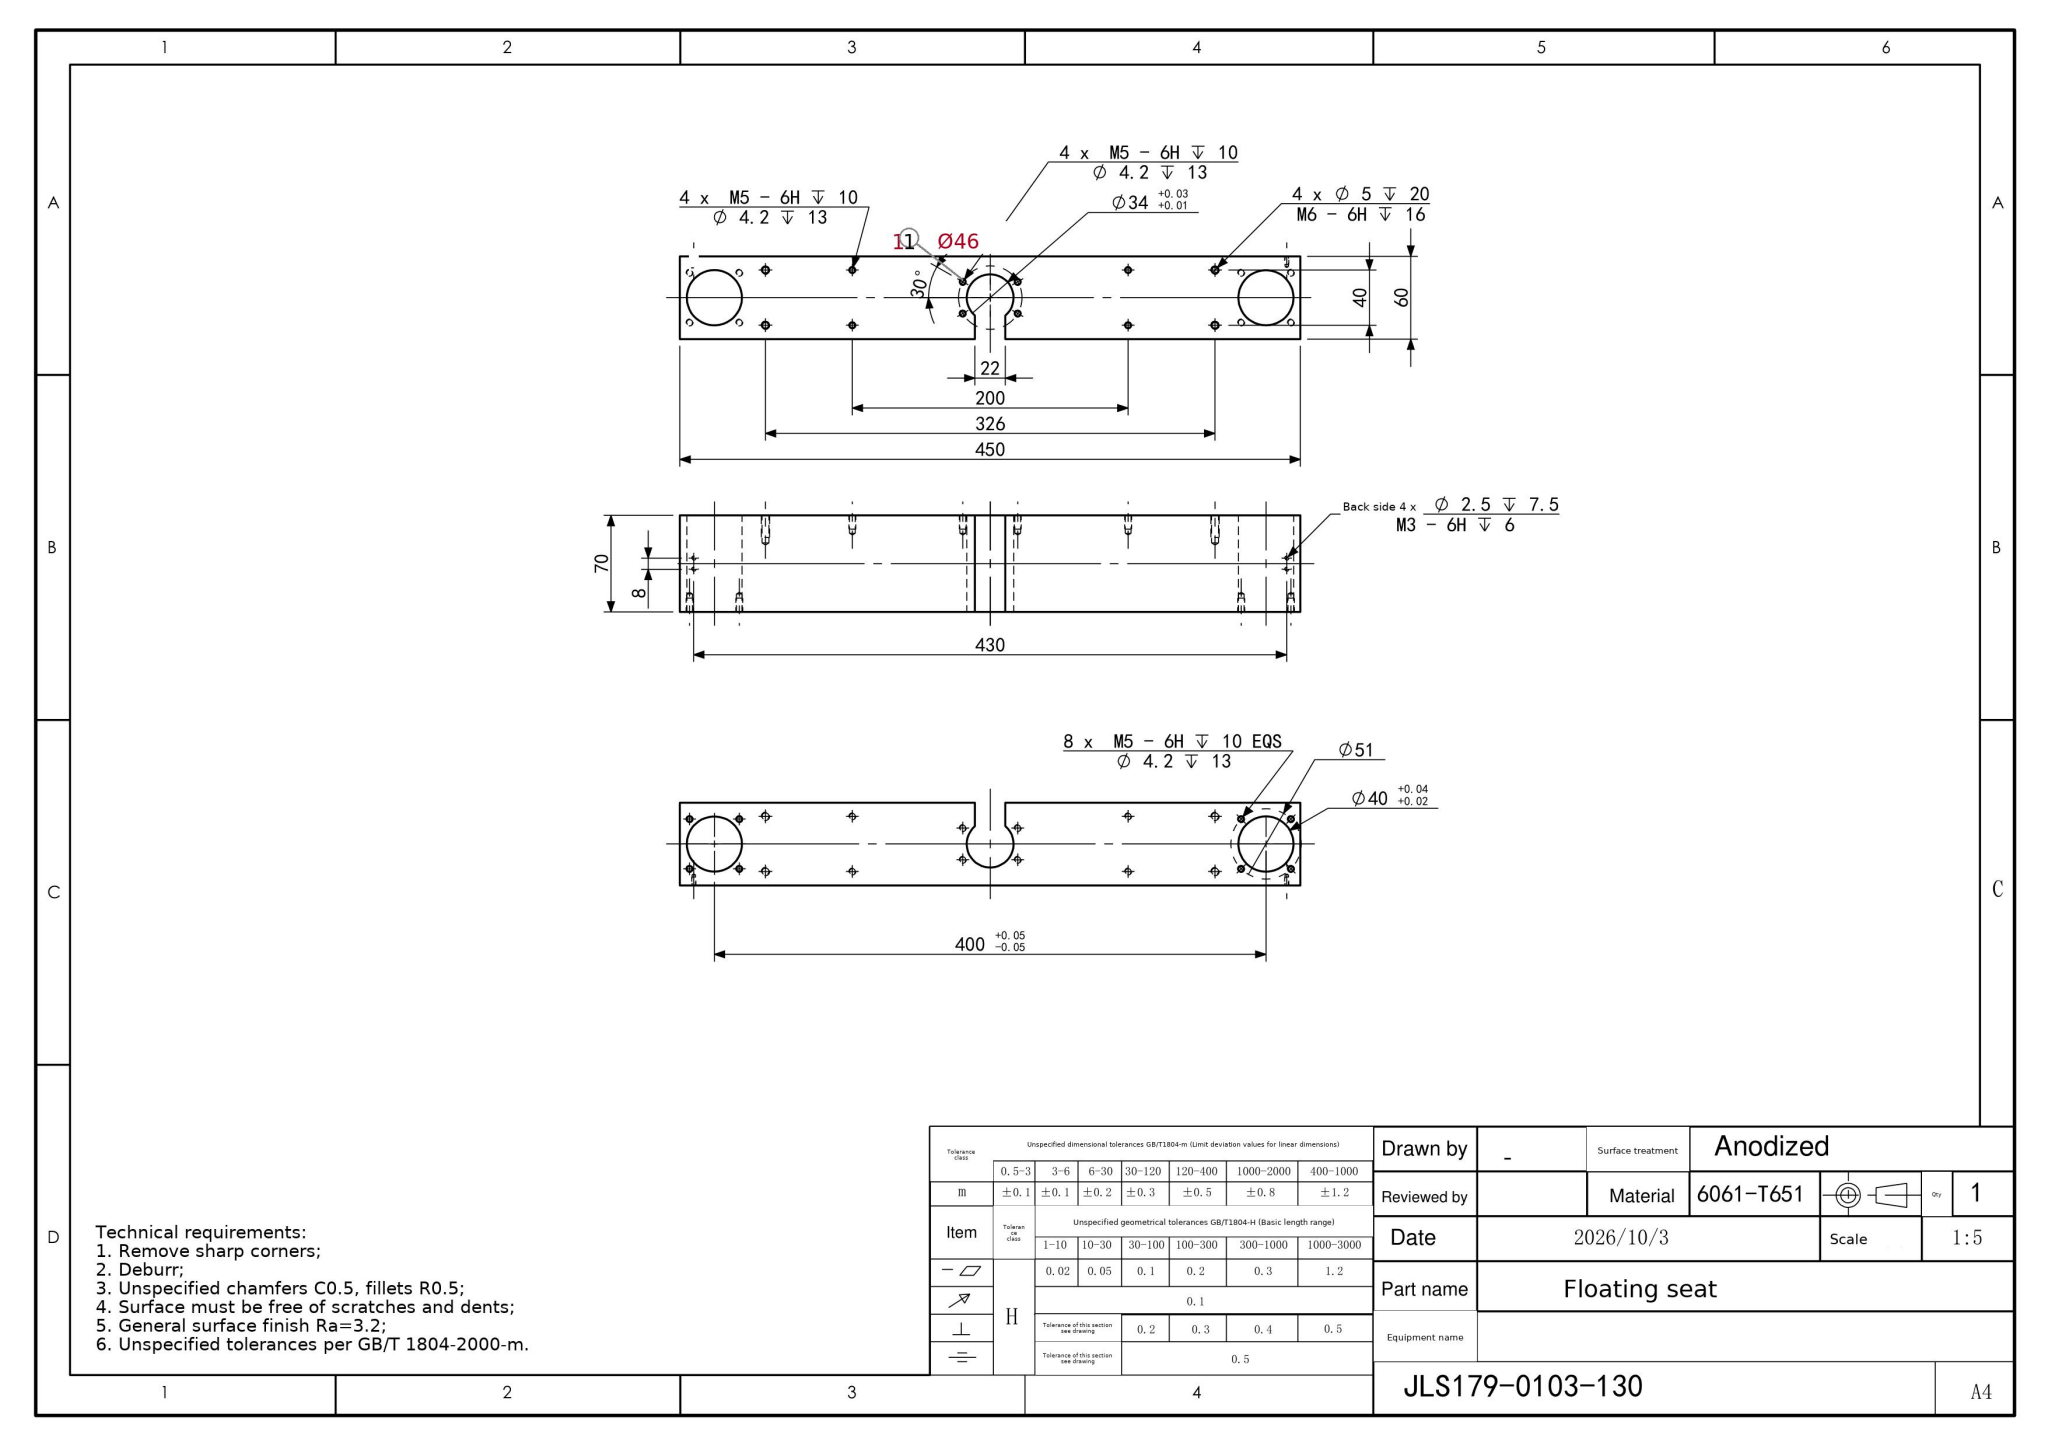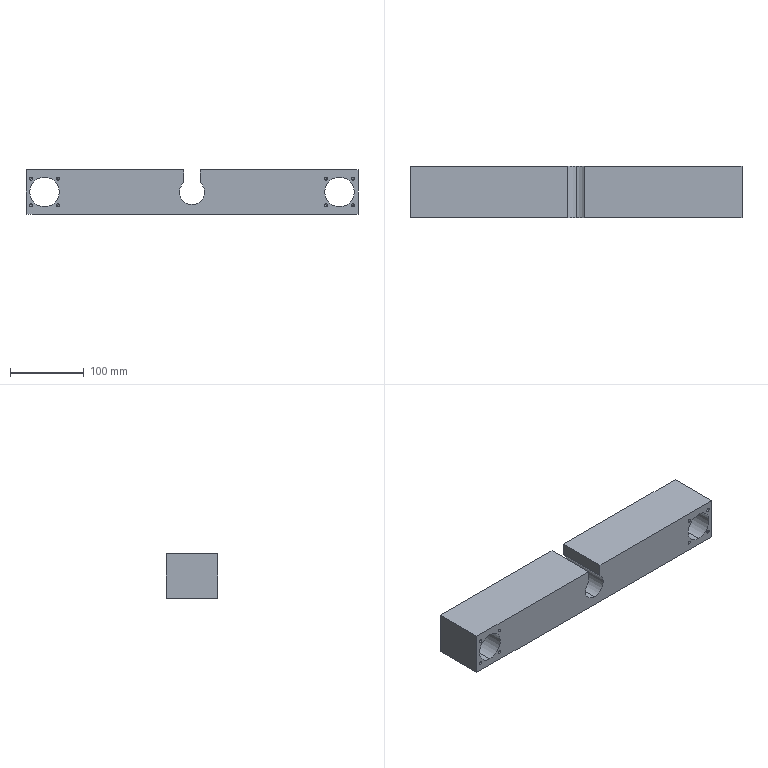Part | SolidWorks | mm | material 6061-T651 | 1 solid | 111 faces | box 450 x 70 x 60 mm | volume 1623796 mm3 | cylinder 54 | cone 48 | plane 9 | commonest cylinder face diameters 4.2 x32 2.5 x8 5 x8 40 x4 34 x2
build123d program:
from build123d import *

# Parameters (mm, degrees)
SKETCH1_W                  = 450
SKETCH1_H                  = 60
SKETCH1_R                  = 20
SKETCH1_R_2                = 17
BOSS_EXTRUDE1_DEPTH        = 35
M5_TAPPED_HOLE1_D          = 4.2
M5_TAPPED_HOLE1_DEPTH      = 13
M5_TAPPED_HOLE1_TIP        = 1.262
M6_TAPPED_HOLE2_D          = 5
M6_TAPPED_HOLE2_DEPTH      = 20
M6_TAPPED_HOLE2_TIP        = 1.502
M3_TAPPED_HOLE1_AT_2_COUNT = 2
M3_TAPPED_HOLE1_AT_2_PITCH = 8
SKETCH14_W                 = 22
SKETCH14_H                 = 121.424
CUT_EXTRUDE1_DEPTH         = 20
M5_TAPPED_HOLE2_D          = 4.2
M5_TAPPED_HOLE2_DEPTH      = 13
M5_TAPPED_HOLE2_TIP        = 1.262
M5_TAPPED_HOLE3_D          = 4.2
M5_TAPPED_HOLE3_DEPTH      = 13
M5_TAPPED_HOLE3_TIP        = 1.262


with BuildPart() as part:
    # Sketch1 → Boss-Extrude1 (new, symmetric)
    with BuildSketch(Plane(origin=(0, 0, 0), x_dir=(1, 0, 0), z_dir=(0, 1, 0))):
        Rectangle(SKETCH1_W, SKETCH1_H)
        with Locations(Location((200, 0, 0), (0, 0, 270))):
            Circle(SKETCH1_R, mode=Mode.SUBTRACT)
        with Locations(Location((-200, 0, 0), (0, 0, 90))):
            Circle(SKETCH1_R, mode=Mode.SUBTRACT)
        with Locations(Location((0, 0, 0), (0, 0, 270))):
            Circle(SKETCH1_R_2, mode=Mode.SUBTRACT)
    extrude(amount=BOSS_EXTRUDE1_DEPTH, both=True)

    # M5 Tapped Hole1
    with Locations(Plane(origin=(0, -35, 0), x_dir=(-1, 0, 0), z_dir=(0, -1, 0))):
        with Locations((218.031, 18.031), (181.969, -18.031), (218.031, -18.031), (181.969, 18.031), (-181.969, 18.031), (-218.031, -18.031), (-181.969, -18.031), (-218.031, 18.031)):
            Hole(M5_TAPPED_HOLE1_D / 2, depth=M5_TAPPED_HOLE1_DEPTH)
            with Locations((0, 0, -(M5_TAPPED_HOLE1_DEPTH + M5_TAPPED_HOLE1_TIP / 2))):  # 118° drill point
                Cone(0, M5_TAPPED_HOLE1_D / 2, M5_TAPPED_HOLE1_TIP, mode=Mode.SUBTRACT)

    # M6 Tapped Hole2
    with Locations(Plane(origin=(0, 35, 0), x_dir=(1, 0, 0), z_dir=(0, 1, 0))):
        with Locations((163, -20), (163, 20), (-163, -20), (-163, 20)):
            Hole(M6_TAPPED_HOLE2_D / 2, depth=M6_TAPPED_HOLE2_DEPTH)
            with Locations((0, 0, -(M6_TAPPED_HOLE2_DEPTH + M6_TAPPED_HOLE2_TIP / 2))):  # 118° drill point
                Cone(0, M6_TAPPED_HOLE2_D / 2, M6_TAPPED_HOLE2_TIP, mode=Mode.SUBTRACT)

    # Sketch9 → M3 Tapped Hole1 (revolve, cut)
    with BuildSketch(Plane(origin=(-215, 4, -30), x_dir=(0, 1, 0), z_dir=(1, 0, 0))):
        Polygon((0, 0), (0, 8.251), (1.25, 7.5), (1.25, 0), align=None)
    m3_tapped_hole1 = revolve(axis=Axis((-215, 4, -36.35), (0, 0, 1)), mode=Mode.SUBTRACT)

    # M3 Tapped Hole1 at 2: M3 Tapped Hole1 ×2
    with Locations(*[(0, -i * M3_TAPPED_HOLE1_AT_2_PITCH, 0) for i in range(1, M3_TAPPED_HOLE1_AT_2_COUNT)]):
        add(m3_tapped_hole1, mode=Mode.SUBTRACT)

    # Mirror1: M3 Tapped Hole1 across plane
    add(m3_tapped_hole1.mirror(Plane(origin=(0, 0, 0), x_dir=(0, 0, 1), z_dir=(1, 0, 0))), mode=Mode.SUBTRACT)

    # Mirror1 copy 1 sketch → Mirror1 copy 1 (revolve, cut)
    with BuildSketch(Plane(origin=(215, -4, -30), x_dir=(0, 1, 0), z_dir=(-1, 0, 0))):
        Polygon((0, 0), (0, -8.251), (1.25, -7.5), (1.25, 0), align=None)
    revolve(axis=Axis((215, -4, -36.35), (0, 0, -1)), mode=Mode.SUBTRACT)

    # Sketch14 → Cut-Extrude1 (cut)
    with BuildSketch(Plane(origin=(0, 0, 30), x_dir=(-1, 0, 0), z_dir=(0, 0, -1))):
        Rectangle(SKETCH14_W, SKETCH14_H)
    extrude(amount=CUT_EXTRUDE1_DEPTH, mode=Mode.SUBTRACT)

    # M5 Tapped Hole2
    with Locations(Plane(origin=(0, 35, 0), x_dir=(1, 0, 0), z_dir=(0, 1, 0))):
        with Locations((-100, -20), (-100, 20), (100, -20), (100, 20)):
            Hole(M5_TAPPED_HOLE2_D / 2, depth=M5_TAPPED_HOLE2_DEPTH)
            with Locations((0, 0, -(M5_TAPPED_HOLE2_DEPTH + M5_TAPPED_HOLE2_TIP / 2))):  # 118° drill point
                Cone(0, M5_TAPPED_HOLE2_D / 2, M5_TAPPED_HOLE2_TIP, mode=Mode.SUBTRACT)

    # M5 Tapped Hole3
    with Locations(Plane(origin=(0, 35, 0), x_dir=(1, 0, 0), z_dir=(0, 1, 0))):
        with Locations((-19.919, -11.5), (19.919, 11.5), (-19.919, 11.5), (19.919, -11.5)):
            Hole(M5_TAPPED_HOLE3_D / 2, depth=M5_TAPPED_HOLE3_DEPTH)
            with Locations((0, 0, -(M5_TAPPED_HOLE3_DEPTH + M5_TAPPED_HOLE3_TIP / 2))):  # 118° drill point
                Cone(0, M5_TAPPED_HOLE3_D / 2, M5_TAPPED_HOLE3_TIP, mode=Mode.SUBTRACT)


solid = part.part